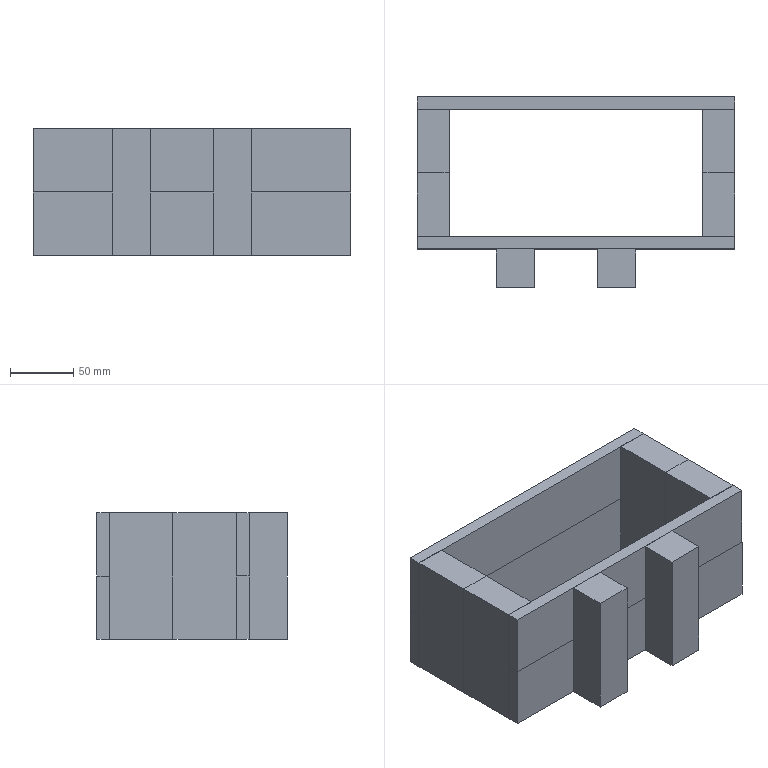Assembly | NX | mm | 10 component files | 10 solids | 60 faces | box 250 x 150 x 100 mm | volume 1180000 mm3 | plane 60
Bill of materials:
unnamed part 1 | 4 |  | Long, thin, flat rectangular bar (a strip-like rectangular prism) with sharp edges and no visible holes, slots or cut-outs.
unnamed part 2 | 2 |  | Rectangular prism with a square cross-section, about 3 to 3.5 times as long as its side width. Plain block or bar with no visible features.
unnamed part 3 | 4 |  | Solid rectangular block (cuboid) with three different edge lengths, in proportions of roughly 1:2:4. No visible features.
Mates:
1. touch align | Front_block 3 edge | Front_block 4 edge
2. touch align | Front_block 4 edge | Front_block 3 edge
3. fix | Front_block 4 component
4. touch align | Front_block 2 edge | Front_block 1 edge
5. touch align | Front_block 2 edge | Front_block 1 edge
6. touch align | front_up 1 face | Front_block 3 face
7. distance | front_up 1 face | Front_block 3 face
8. touch align | front_up 1 face | Front_block 3 face
9. touch align | front_up 2 face | Front_block 3 face
10. distance | front_up 2 face | front_up 1 face
11. touch align | front_up 2 face | Front_block 3 face
12. touch align | Front_block 3 face | Front_block 2 face
13. touch align | Front_block 3 face | Front_block 2 face
14. distance | Front_block 3 face | Front_block 2 face
15. touch align | side 4 edge | Front_block 3 edge
16. touch align | side 4 face | Front_block 3 face
17. touch align | side 4 face | Front_block 4 face
18. touch align | side 3 edge | side 4 edge
19. touch align | side 3 face | side 4 face
20. touch align | Front_block 2 face | side 3 face
21. touch align | side 2 face | Front_block 2 face
22. touch align | side 2 face | Front_block 2 face
23. touch align | side 2 face | Front_block 2 face
24. touch align | side 1 face | side 2 face
25. touch align | side 1 face | side 2 face
26. touch align | side 1 face | Front_block 3 face
27. touch align | side 1 face | Front_block 3 face